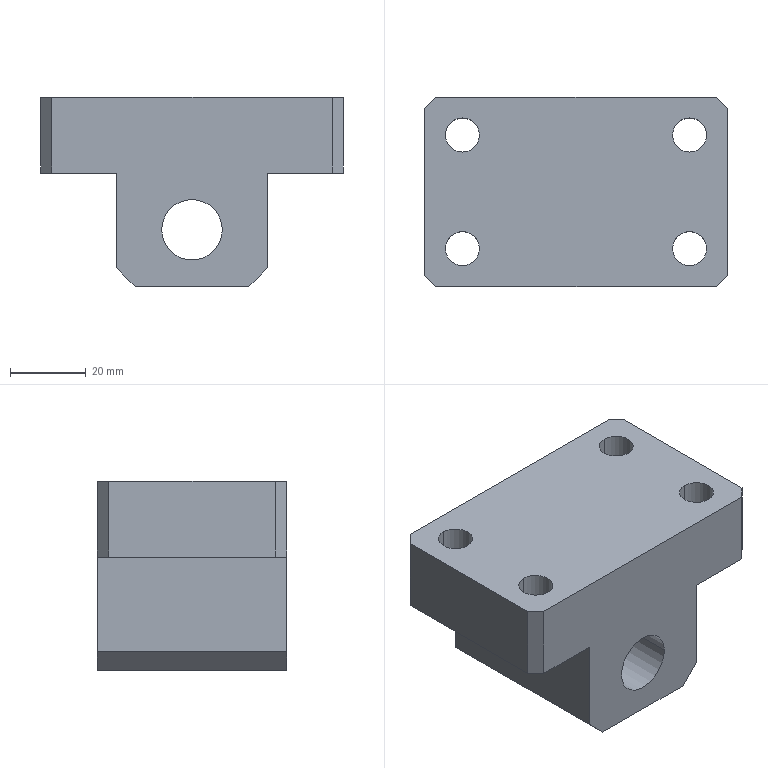Component | SolidWorks | -CylinderConnectionSeat-1 | 1 solid | 38 faces | box 80 x 50 x 50 mm | volume 120357 mm3 | plane 20 | cylinder 18 | commonest cylinder face diameters 14 x8 9 x8 16 x2
build123d program:
from build123d import *

# Parameters (mm, degrees)
EXTRUDE1_DEPTH                                      = 50
M16X1_5_TAPPED_HOLE1_D                              = 16
CHAMFER1_SIZE                                       = 5
CYLINDRICAL_COUNTERSUNK_HOLE_FOR_M8_HEX_D           = 9
CYLINDRICAL_COUNTERSUNK_HOLE_FOR_M8_HEX_CBORE_D     = 14
CYLINDRICAL_COUNTERSUNK_HOLE_FOR_M8_HEX_CBORE_DEPTH = 8
CHAMFER2_SIZE                                       = 3


with BuildPart() as part:
    # Sketch1 → Extrude1 (new body)
    with BuildSketch(Plane.XY):
        Polygon((-40, 25), (40, 25), (40, 5), (20, 5), (20, -25), (-20, -25), (-20, 5), (-40, 5), align=None)
    extrude(amount=EXTRUDE1_DEPTH)

    # M16x1.5 Tapped Hole1 (through all)
    with Locations(Plane.XY.offset(50)):
        with Locations((0, -10)):
            Hole(M16X1_5_TAPPED_HOLE1_D / 2)

    # Chamfer1
    chamfer1_edges = [part.edges().sort_by_distance(p)[0] for p in [
        (20, -25, 25),
        (-20, -25, 25),
    ]]
    chamfer(chamfer1_edges, length=CHAMFER1_SIZE)

    # Cylindrical Countersunk Hole for M8 Hex (through all)
    with Locations(Plane.XZ.offset(-5)):
        with Locations((-30, 40), (-30, 10), (30, 40), (30, 10)):
            CounterBoreHole(CYLINDRICAL_COUNTERSUNK_HOLE_FOR_M8_HEX_D / 2, CYLINDRICAL_COUNTERSUNK_HOLE_FOR_M8_HEX_CBORE_D / 2, CYLINDRICAL_COUNTERSUNK_HOLE_FOR_M8_HEX_CBORE_DEPTH)

    # Chamfer2
    chamfer2_edges = [part.edges().sort_by_distance(p)[0] for p in [
        (-40, 15, 0),
        (40, 15, 50),
        (-40, 15, 50),
        (40, 15, 0),
    ]]
    chamfer(chamfer2_edges, length=CHAMFER2_SIZE)


solid = part.part

# Placed as in the assembly
solid = solid.moved(Location((30, 1289.5, -110), (90, 0, 0)))